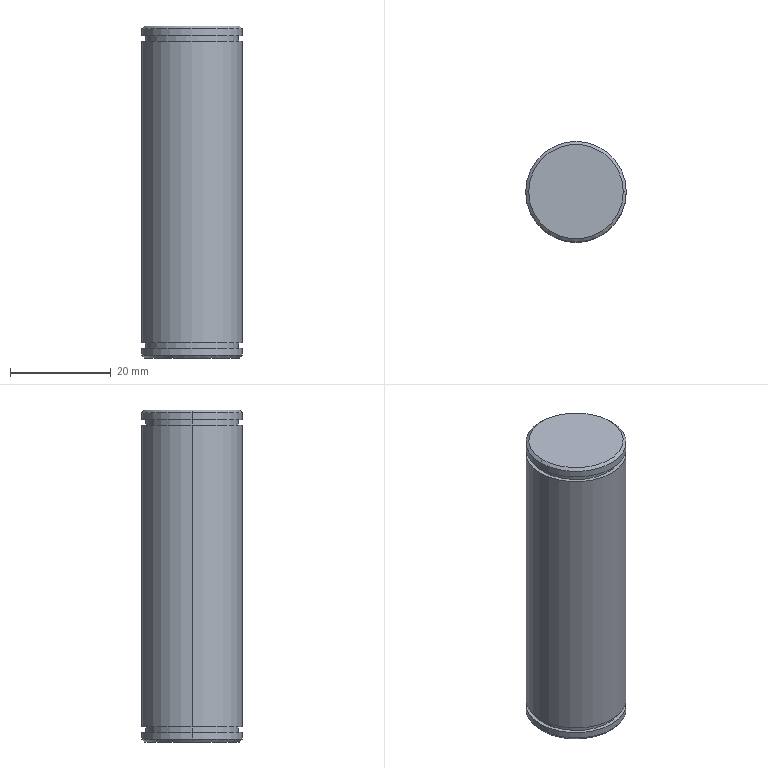Component | SolidWorks | ConnectingPin1-1 | 1 solid | 20 faces | box 20 x 20 x 66 mm | volume 20616 mm3 | cylinder 10 | plane 6 | cone 4 | commonest cylinder face diameters 20 x6 18.5 x4
build123d program:
from build123d import *
from OCP.BRepFilletAPI import BRepFilletAPI_MakeChamfer

# Parameters (mm, degrees)
SKETCH1_R           = 10
BOSS_EXTRUDE1_DEPTH = 33
CHAMFER1_SIZE       = 0.5
CHAMFER1_SIZE2      = 0.5959
SKETCH3_W           = 0.75
SKETCH3_H           = 1.1


with BuildPart() as part:
    # Sketch1 → Boss-Extrude1 (new, symmetric)
    with BuildSketch(Plane.XY):
        Circle(SKETCH1_R)
    extrude(amount=BOSS_EXTRUDE1_DEPTH, both=True)

    # Chamfer1: one chamfer whose edges measure the first distance from different faces: ONE call of the kernel's chamfer builder (chamfer() names one face for all edges)
    chamfer1_edges_1 = [part.edges().sort_by_distance(p)[0] for p in [
        (-10, 0, -33),
    ]]
    chamfer1_side_1 = [part.faces().sort_by_distance(p)[0] for p in [
        (0, 0, -33),
    ]]
    chamfer1_edges_2 = [part.edges().sort_by_distance(p)[0] for p in [
        (-10, 0, 33),
    ]]
    chamfer1_side_2 = [part.faces().sort_by_distance(p)[0] for p in [
        (-10, 0, 0),
    ]]
    chamfer1 = BRepFilletAPI_MakeChamfer(part.part.solid().wrapped)
    for e in chamfer1_edges_1:
        chamfer1.Add(CHAMFER1_SIZE, CHAMFER1_SIZE2, e.wrapped, chamfer1_side_1[0].wrapped)  # the first distance lies on this face
    for e in chamfer1_edges_2:
        chamfer1.Add(CHAMFER1_SIZE, CHAMFER1_SIZE2, e.wrapped, chamfer1_side_2[0].wrapped)  # the first distance lies on this face
    add(Compound.cast(chamfer1.Shape()), mode=Mode.REPLACE)

    # Sketch3 → Cut-Revolve1 (revolve, cut)
    with BuildSketch(Plane(origin=(0, 0, 0), x_dir=(1, 0, 0), z_dir=(0, 1, 0))):
        with Locations((9.625, -30.55)):
            Rectangle(SKETCH3_W, SKETCH3_H)
    cut_revolve1 = revolve(axis=Axis((0, 0, 33), (0, 0, -1)), mode=Mode.SUBTRACT)

    # Mirror2: Cut-Revolve1 across plane
    add(cut_revolve1.mirror(Plane.XY), mode=Mode.SUBTRACT)


solid = part.part

# Placed as in the assembly
solid = solid.moved(Location((-372.766, -43.543, 900), (0, 0, 0)))
STEP:
#1=COLOUR_RGB('',0.7922,0.8196,0.9333);
#2=FILL_AREA_STYLE_COLOUR('',#1);
#3=FILL_AREA_STYLE('',(#2));
#4=SURFACE_STYLE_FILL_AREA(#3);
#5=SURFACE_SIDE_STYLE('',(#4));
#6=SURFACE_STYLE_USAGE(.BOTH.,#5);
#7=PRESENTATION_STYLE_ASSIGNMENT((#6));
#8=CARTESIAN_POINT('',(-14.282,-1.714,34.209));
#9=VERTEX_POINT('',#8);
#10=CARTESIAN_POINT('',(-15.07,-1.714,34.209));
#11=VERTEX_POINT('',#10);
#12=CARTESIAN_POINT('',(-14.676,-1.714,34.209));
#13=DIRECTION('',(0.,-0.,1.));
#14=DIRECTION('',(1.,0.,0.));
#15=AXIS2_PLACEMENT_3D('',#12,#13,#14);
#16=CIRCLE('',#15,0.3937);
#17=EDGE_CURVE('',#9,#11,#16,.T.);
#18=ORIENTED_EDGE('',*,*,#17,.F.);
#19=CARTESIAN_POINT('',(-14.282,-1.714,34.157));
#20=VERTEX_POINT('',#19);
#21=CARTESIAN_POINT('',(-14.282,-1.714,36.732));
#22=DIRECTION('',(-0.,0.,-1.));
#23=VECTOR('',#22,39.37);
#24=LINE('',#21,#23);
#25=EDGE_CURVE('',#9,#20,#24,.T.);
#26=ORIENTED_EDGE('',*,*,#25,.T.);
#27=CARTESIAN_POINT('',(-15.07,-1.714,34.157));
#28=VERTEX_POINT('',#27);
#29=CARTESIAN_POINT('',(-14.676,-1.714,34.157));
#30=DIRECTION('',(0.,-0.,1.));
#31=DIRECTION('',(1.,0.,0.));
#32=AXIS2_PLACEMENT_3D('',#29,#30,#31);
#33=CIRCLE('',#32,0.3937);
#34=EDGE_CURVE('',#20,#28,#33,.T.);
#35=ORIENTED_EDGE('',*,*,#34,.T.);
#36=CARTESIAN_POINT('',(-15.07,-1.714,36.732));
#37=DIRECTION('',(-0.,0.,-1.));
#38=VECTOR('',#37,39.37);
#39=LINE('',#36,#38);
#40=EDGE_CURVE('',#11,#28,#39,.T.);
#41=ORIENTED_EDGE('',*,*,#40,.F.);
#42=EDGE_LOOP('',(#18,#26,#35,#41));
#43=FACE_OUTER_BOUND('',#42,.T.);
#44=CARTESIAN_POINT('',(-14.676,-1.714,36.732));
#45=DIRECTION('',(-0.,0.,-1.));
#46=DIRECTION('',(-1.,-0.,0.));
#47=AXIS2_PLACEMENT_3D('',#44,#45,#46);
#48=CYLINDRICAL_SURFACE('',#47,0.3937);
#49=ADVANCED_FACE('',(#43),#48,.T.);
#50=CARTESIAN_POINT('',(-15.05,-1.714,34.134));
#51=VERTEX_POINT('',#50);
#52=CARTESIAN_POINT('',(-14.302,-1.714,34.134));
#53=VERTEX_POINT('',#52);
#54=CARTESIAN_POINT('',(-14.676,-1.714,34.134));
#55=DIRECTION('',(-0.,0.,-1.));
#56=DIRECTION('',(1.,0.,0.));
#57=AXIS2_PLACEMENT_3D('',#54,#55,#56);
#58=CIRCLE('',#57,0.374);
#59=EDGE_CURVE('',#51,#53,#58,.T.);
#60=ORIENTED_EDGE('',*,*,#59,.F.);
#61=CARTESIAN_POINT('',(-15.07,-1.714,34.157));
#62=DIRECTION('',(-0.6428,-0.,0.766));
#63=VECTOR('',#62,39.37);
#64=LINE('',#61,#63);
#65=EDGE_CURVE('',#51,#28,#64,.T.);
#66=ORIENTED_EDGE('',*,*,#65,.T.);
#67=ORIENTED_EDGE('',*,*,#34,.F.);
#68=CARTESIAN_POINT('',(-14.282,-1.714,34.157));
#69=DIRECTION('',(0.6428,0.,0.766));
#70=VECTOR('',#69,39.37);
#71=LINE('',#68,#70);
#72=EDGE_CURVE('',#53,#20,#71,.T.);
#73=ORIENTED_EDGE('',*,*,#72,.F.);
#74=EDGE_LOOP('',(#60,#66,#67,#73));
#75=FACE_OUTER_BOUND('',#74,.T.);
#76=CARTESIAN_POINT('',(-14.676,-1.714,34.157));
#77=DIRECTION('',(0.,-0.,1.));
#78=DIRECTION('',(1.,0.,0.));
#79=AXIS2_PLACEMENT_3D('',#76,#77,#78);
#80=CONICAL_SURFACE('',#79,0.3937,0.6981);
#81=ADVANCED_FACE('',(#75),#80,.T.);
#82=CARTESIAN_POINT('',(-15.04,-1.714,34.252));
#83=VERTEX_POINT('',#82);
#84=CARTESIAN_POINT('',(-14.312,-1.714,34.252));
#85=VERTEX_POINT('',#84);
#86=CARTESIAN_POINT('',(-14.676,-1.714,34.252));
#87=DIRECTION('',(0.,-0.,1.));
#88=DIRECTION('',(1.,0.,0.));
#89=AXIS2_PLACEMENT_3D('',#86,#87,#88);
#90=CIRCLE('',#89,0.3642);
#91=EDGE_CURVE('',#83,#85,#90,.T.);
#92=ORIENTED_EDGE('',*,*,#91,.F.);
#93=CARTESIAN_POINT('',(-15.04,-1.714,34.209));
#94=VERTEX_POINT('',#93);
#95=CARTESIAN_POINT('',(-15.04,-1.714,34.252));
#96=DIRECTION('',(-0.,0.,-1.));
#97=VECTOR('',#96,39.37);
#98=LINE('',#95,#97);
#99=EDGE_CURVE('',#83,#94,#98,.T.);
#100=ORIENTED_EDGE('',*,*,#99,.T.);
#101=CARTESIAN_POINT('',(-14.312,-1.714,34.209));
#102=VERTEX_POINT('',#101);
#103=CARTESIAN_POINT('',(-14.676,-1.714,34.209));
#104=DIRECTION('',(0.,-0.,1.));
#105=DIRECTION('',(1.,0.,0.));
#106=AXIS2_PLACEMENT_3D('',#103,#104,#105);
#107=CIRCLE('',#106,0.3642);
#108=EDGE_CURVE('',#94,#102,#107,.T.);
#109=ORIENTED_EDGE('',*,*,#108,.T.);
#110=CARTESIAN_POINT('',(-14.312,-1.714,34.252));
#111=DIRECTION('',(-0.,0.,-1.));
#112=VECTOR('',#111,39.37);
#113=LINE('',#110,#112);
#114=EDGE_CURVE('',#85,#102,#113,.T.);
#115=ORIENTED_EDGE('',*,*,#114,.F.);
#116=EDGE_LOOP('',(#92,#100,#109,#115));
#117=FACE_OUTER_BOUND('',#116,.T.);
#118=CARTESIAN_POINT('',(-14.676,-1.714,34.252));
#119=DIRECTION('',(-0.,0.,-1.));
#120=DIRECTION('',(1.,0.,0.));
#121=AXIS2_PLACEMENT_3D('',#118,#119,#120);
#122=CYLINDRICAL_SURFACE('',#121,0.3642);
#123=ADVANCED_FACE('',(#117),#122,.T.);
#124=CARTESIAN_POINT('',(-15.07,-1.714,36.713));
#125=VERTEX_POINT('',#124);
#126=CARTESIAN_POINT('',(-14.282,-1.714,36.713));
#127=VERTEX_POINT('',#126);
#128=CARTESIAN_POINT('',(-14.676,-1.714,36.713));
#129=DIRECTION('',(-0.,0.,-1.));
#130=DIRECTION('',(1.,0.,0.));
#131=AXIS2_PLACEMENT_3D('',#128,#129,#130);
#132=CIRCLE('',#131,0.3937);
#133=EDGE_CURVE('',#125,#127,#132,.T.);
#134=ORIENTED_EDGE('',*,*,#133,.T.);
#135=CARTESIAN_POINT('',(-14.282,-1.714,36.657));
#136=VERTEX_POINT('',#135);
#137=CARTESIAN_POINT('',(-14.282,-1.714,36.732));
#138=DIRECTION('',(-0.,0.,-1.));
#139=VECTOR('',#138,39.37);
#140=LINE('',#137,#139);
#141=EDGE_CURVE('',#127,#136,#140,.T.);
#142=ORIENTED_EDGE('',*,*,#141,.T.);
#143=CARTESIAN_POINT('',(-15.07,-1.714,36.657));
#144=VERTEX_POINT('',#143);
#145=CARTESIAN_POINT('',(-14.676,-1.714,36.657));
#146=DIRECTION('',(0.,-0.,1.));
#147=DIRECTION('',(1.,0.,0.));
#148=AXIS2_PLACEMENT_3D('',#145,#146,#147);
#149=CIRCLE('',#148,0.3937);
#150=EDGE_CURVE('',#136,#144,#149,.T.);
#151=ORIENTED_EDGE('',*,*,#150,.T.);
#152=CARTESIAN_POINT('',(-15.07,-1.714,36.732));
#153=DIRECTION('',(-0.,0.,-1.));
#154=VECTOR('',#153,39.37);
#155=LINE('',#152,#154);
#156=EDGE_CURVE('',#125,#144,#155,.T.);
#157=ORIENTED_EDGE('',*,*,#156,.F.);
#158=EDGE_LOOP('',(#134,#142,#151,#157));
#159=FACE_OUTER_BOUND('',#158,.T.);
#160=CARTESIAN_POINT('',(-14.676,-1.714,36.732));
#161=DIRECTION('',(-0.,0.,-1.));
#162=DIRECTION('',(-1.,-0.,0.));
#163=AXIS2_PLACEMENT_3D('',#160,#161,#162);
#164=CYLINDRICAL_SURFACE('',#163,0.3937);
#165=ADVANCED_FACE('',(#159),#164,.T.);
#166=CARTESIAN_POINT('',(-14.306,-1.714,36.732));
#167=VERTEX_POINT('',#166);
#168=CARTESIAN_POINT('',(-15.046,-1.714,36.732));
#169=VERTEX_POINT('',#168);
#170=CARTESIAN_POINT('',(-14.676,-1.714,36.732));
#171=DIRECTION('',(0.,-0.,1.));
#172=DIRECTION('',(1.,0.,0.));
#173=AXIS2_PLACEMENT_3D('',#170,#171,#172);
#174=CIRCLE('',#173,0.3702);
#175=EDGE_CURVE('',#167,#169,#174,.T.);
#176=ORIENTED_EDGE('',*,*,#175,.F.);
#177=CARTESIAN_POINT('',(-14.306,-1.714,36.732));
#178=DIRECTION('',(0.766,0.,-0.6428));
#179=VECTOR('',#178,39.37);
#180=LINE('',#177,#179);
#181=EDGE_CURVE('',#167,#127,#180,.T.);
#182=ORIENTED_EDGE('',*,*,#181,.T.);
#183=ORIENTED_EDGE('',*,*,#133,.F.);
#184=CARTESIAN_POINT('',(-15.046,-1.714,36.732));
#185=DIRECTION('',(-0.766,-0.,-0.6428));
#186=VECTOR('',#185,39.37);
#187=LINE('',#184,#186);
#188=EDGE_CURVE('',#169,#125,#187,.T.);
#189=ORIENTED_EDGE('',*,*,#188,.F.);
#190=EDGE_LOOP('',(#176,#182,#183,#189));
#191=FACE_OUTER_BOUND('',#190,.T.);
#192=CARTESIAN_POINT('',(-14.676,-1.714,36.732));
#193=DIRECTION('',(-0.,0.,-1.));
#194=DIRECTION('',(-1.,-0.,0.));
#195=AXIS2_PLACEMENT_3D('',#192,#193,#194);
#196=CONICAL_SURFACE('',#195,0.3702,0.8727);
#197=ADVANCED_FACE('',(#191),#196,.T.);
#198=CARTESIAN_POINT('',(-14.312,-1.714,36.614));
#199=VERTEX_POINT('',#198);
#200=CARTESIAN_POINT('',(-15.04,-1.714,36.614));
#201=VERTEX_POINT('',#200);
#202=CARTESIAN_POINT('',(-14.676,-1.714,36.614));
#203=DIRECTION('',(0.,-0.,1.));
#204=DIRECTION('',(1.,0.,0.));
#205=AXIS2_PLACEMENT_3D('',#202,#203,#204);
#206=CIRCLE('',#205,0.3642);
#207=EDGE_CURVE('',#199,#201,#206,.T.);
#208=ORIENTED_EDGE('',*,*,#207,.T.);
#209=CARTESIAN_POINT('',(-15.04,-1.714,36.657));
#210=VERTEX_POINT('',#209);
#211=CARTESIAN_POINT('',(-15.04,-1.714,36.713));
#212=DIRECTION('',(0.,-0.,1.));
#213=VECTOR('',#212,39.37);
#214=LINE('',#211,#213);
#215=EDGE_CURVE('',#201,#210,#214,.T.);
#216=ORIENTED_EDGE('',*,*,#215,.T.);
#217=CARTESIAN_POINT('',(-14.312,-1.714,36.657));
#218=VERTEX_POINT('',#217);
#219=CARTESIAN_POINT('',(-14.676,-1.714,36.657));
#220=DIRECTION('',(0.,-0.,1.));
#221=DIRECTION('',(1.,0.,0.));
#222=AXIS2_PLACEMENT_3D('',#219,#220,#221);
#223=CIRCLE('',#222,0.3642);
#224=EDGE_CURVE('',#218,#210,#223,.T.);
#225=ORIENTED_EDGE('',*,*,#224,.F.);
#226=CARTESIAN_POINT('',(-14.312,-1.714,36.713));
#227=DIRECTION('',(0.,-0.,1.));
#228=VECTOR('',#227,39.37);
#229=LINE('',#226,#228);
#230=EDGE_CURVE('',#199,#218,#229,.T.);
#231=ORIENTED_EDGE('',*,*,#230,.F.);
#232=EDGE_LOOP('',(#208,#216,#225,#231));
#233=FACE_OUTER_BOUND('',#232,.T.);
#234=CARTESIAN_POINT('',(-14.676,-1.714,36.713));
#235=DIRECTION('',(0.,-0.,1.));
#236=DIRECTION('',(1.,0.,0.));
#237=AXIS2_PLACEMENT_3D('',#234,#235,#236);
#238=CYLINDRICAL_SURFACE('',#237,0.3642);
#239=ADVANCED_FACE('',(#233),#238,.T.);
#240=CARTESIAN_POINT('',(-14.282,-1.714,36.614));
#241=VERTEX_POINT('',#240);
#242=CARTESIAN_POINT('',(-15.07,-1.714,36.614));
#243=VERTEX_POINT('',#242);
#244=CARTESIAN_POINT('',(-14.676,-1.714,36.614));
#245=DIRECTION('',(0.,-0.,1.));
#246=DIRECTION('',(1.,0.,0.));
#247=AXIS2_PLACEMENT_3D('',#244,#245,#246);
#248=CIRCLE('',#247,0.3937);
#249=EDGE_CURVE('',#241,#243,#248,.T.);
#250=ORIENTED_EDGE('',*,*,#249,.F.);
#251=CARTESIAN_POINT('',(-14.282,-1.714,34.252));
#252=VERTEX_POINT('',#251);
#253=CARTESIAN_POINT('',(-14.282,-1.714,36.732));
#254=DIRECTION('',(-0.,0.,-1.));
#255=VECTOR('',#254,39.37);
#256=LINE('',#253,#255);
#257=EDGE_CURVE('',#241,#252,#256,.T.);
#258=ORIENTED_EDGE('',*,*,#257,.T.);
#259=CARTESIAN_POINT('',(-15.07,-1.714,34.252));
#260=VERTEX_POINT('',#259);
#261=CARTESIAN_POINT('',(-14.676,-1.714,34.252));
#262=DIRECTION('',(0.,-0.,1.));
#263=DIRECTION('',(1.,0.,0.));
#264=AXIS2_PLACEMENT_3D('',#261,#262,#263);
#265=CIRCLE('',#264,0.3937);
#266=EDGE_CURVE('',#252,#260,#265,.T.);
#267=ORIENTED_EDGE('',*,*,#266,.T.);
#268=CARTESIAN_POINT('',(-15.07,-1.714,36.732));
#269=DIRECTION('',(-0.,0.,-1.));
#270=VECTOR('',#269,39.37);
#271=LINE('',#268,#270);
#272=EDGE_CURVE('',#243,#260,#271,.T.);
#273=ORIENTED_EDGE('',*,*,#272,.F.);
#274=EDGE_LOOP('',(#250,#258,#267,#273));
#275=FACE_OUTER_BOUND('',#274,.T.);
#276=CARTESIAN_POINT('',(-14.676,-1.714,36.732));
#277=DIRECTION('',(-0.,0.,-1.));
#278=DIRECTION('',(-1.,-0.,0.));
#279=AXIS2_PLACEMENT_3D('',#276,#277,#278);
#280=CYLINDRICAL_SURFACE('',#279,0.3937);
#281=ADVANCED_FACE('',(#275),#280,.T.);
#282=ORIENTED_EDGE('',*,*,#257,.F.);
#283=CARTESIAN_POINT('',(-14.676,-1.714,36.614));
#284=DIRECTION('',(0.,-0.,1.));
#285=DIRECTION('',(1.,0.,0.));
#286=AXIS2_PLACEMENT_3D('',#283,#284,#285);
#287=CIRCLE('',#286,0.3937);
#288=EDGE_CURVE('',#243,#241,#287,.T.);
#289=ORIENTED_EDGE('',*,*,#288,.F.);
#290=ORIENTED_EDGE('',*,*,#272,.T.);
#291=CARTESIAN_POINT('',(-14.676,-1.714,34.252));
#292=DIRECTION('',(0.,-0.,1.));
#293=DIRECTION('',(1.,0.,0.));
#294=AXIS2_PLACEMENT_3D('',#291,#292,#293);
#295=CIRCLE('',#294,0.3937);
#296=EDGE_CURVE('',#260,#252,#295,.T.);
#297=ORIENTED_EDGE('',*,*,#296,.T.);
#298=EDGE_LOOP('',(#282,#289,#290,#297));
#299=FACE_OUTER_BOUND('',#298,.T.);
#300=CARTESIAN_POINT('',(-14.676,-1.714,36.732));
#301=DIRECTION('',(-0.,0.,-1.));
#302=DIRECTION('',(-1.,-0.,0.));
#303=AXIS2_PLACEMENT_3D('',#300,#301,#302);
#304=CYLINDRICAL_SURFACE('',#303,0.3937);
#305=ADVANCED_FACE('',(#299),#304,.T.);
#306=ORIENTED_EDGE('',*,*,#207,.F.);
#307=CARTESIAN_POINT('',(-14.676,-1.714,36.614));
#308=DIRECTION('',(0.,-0.,1.));
#309=DIRECTION('',(1.,0.,0.));
#310=AXIS2_PLACEMENT_3D('',#307,#308,#309);
#311=CIRCLE('',#310,0.3642);
#312=EDGE_CURVE('',#201,#199,#311,.T.);
#313=ORIENTED_EDGE('',*,*,#312,.F.);
#314=EDGE_LOOP('',(#306,#313));
#315=FACE_BOUND('',#314,.T.);
#316=ORIENTED_EDGE('',*,*,#288,.T.);
#317=ORIENTED_EDGE('',*,*,#249,.T.);
#318=EDGE_LOOP('',(#316,#317));
#319=FACE_OUTER_BOUND('',#318,.T.);
#320=CARTESIAN_POINT('',(-14.282,-1.714,36.614));
#321=DIRECTION('',(-0.,0.,-1.));
#322=DIRECTION('',(-1.,-0.,0.));
#323=AXIS2_PLACEMENT_3D('',#320,#321,#322);
#324=PLANE('',#323);
#325=ADVANCED_FACE('',(#315,#319),#324,.F.);
#326=ORIENTED_EDGE('',*,*,#215,.F.);
#327=ORIENTED_EDGE('',*,*,#312,.T.);
#328=ORIENTED_EDGE('',*,*,#230,.T.);
#329=CARTESIAN_POINT('',(-14.676,-1.714,36.657));
#330=DIRECTION('',(0.,-0.,1.));
#331=DIRECTION('',(1.,0.,0.));
#332=AXIS2_PLACEMENT_3D('',#329,#330,#331);
#333=CIRCLE('',#332,0.3642);
#334=EDGE_CURVE('',#210,#218,#333,.T.);
#335=ORIENTED_EDGE('',*,*,#334,.F.);
#336=EDGE_LOOP('',(#326,#327,#328,#335));
#337=FACE_OUTER_BOUND('',#336,.T.);
#338=CARTESIAN_POINT('',(-14.676,-1.714,36.713));
#339=DIRECTION('',(0.,-0.,1.));
#340=DIRECTION('',(1.,0.,0.));
#341=AXIS2_PLACEMENT_3D('',#338,#339,#340);
#342=CYLINDRICAL_SURFACE('',#341,0.3642);
#343=ADVANCED_FACE('',(#337),#342,.T.);
#344=CARTESIAN_POINT('',(-14.676,-1.714,36.657));
#345=DIRECTION('',(0.,-0.,1.));
#346=DIRECTION('',(1.,0.,0.));
#347=AXIS2_PLACEMENT_3D('',#344,#345,#346);
#348=CIRCLE('',#347,0.3937);
#349=EDGE_CURVE('',#144,#136,#348,.T.);
#350=ORIENTED_EDGE('',*,*,#349,.F.);
#351=ORIENTED_EDGE('',*,*,#150,.F.);
#352=EDGE_LOOP('',(#350,#351));
#353=FACE_OUTER_BOUND('',#352,.T.);
#354=ORIENTED_EDGE('',*,*,#224,.T.);
#355=ORIENTED_EDGE('',*,*,#334,.T.);
#356=EDGE_LOOP('',(#354,#355));
#357=FACE_BOUND('',#356,.T.);
#358=CARTESIAN_POINT('',(-14.282,-1.714,36.657));
#359=DIRECTION('',(0.,-0.,1.));
#360=DIRECTION('',(1.,0.,-0.));
#361=AXIS2_PLACEMENT_3D('',#358,#359,#360);
#362=PLANE('',#361);
#363=ADVANCED_FACE('',(#353,#357),#362,.F.);
#364=CARTESIAN_POINT('',(-14.676,-1.714,36.732));
#365=DIRECTION('',(0.,-0.,1.));
#366=DIRECTION('',(1.,0.,0.));
#367=AXIS2_PLACEMENT_3D('',#364,#365,#366);
#368=CIRCLE('',#367,0.3702);
#369=EDGE_CURVE('',#169,#167,#368,.T.);
#370=ORIENTED_EDGE('',*,*,#369,.T.);
#371=ORIENTED_EDGE('',*,*,#175,.T.);
#372=EDGE_LOOP('',(#370,#371));
#373=FACE_OUTER_BOUND('',#372,.T.);
#374=CARTESIAN_POINT('',(-14.676,-1.714,36.732));
#375=DIRECTION('',(0.,-0.,1.));
#376=DIRECTION('',(1.,0.,-0.));
#377=AXIS2_PLACEMENT_3D('',#374,#375,#376);
#378=PLANE('',#377);
#379=ADVANCED_FACE('',(#373),#378,.T.);
#380=ORIENTED_EDGE('',*,*,#181,.F.);
#381=ORIENTED_EDGE('',*,*,#369,.F.);
#382=ORIENTED_EDGE('',*,*,#188,.T.);
#383=CARTESIAN_POINT('',(-14.676,-1.714,36.713));
#384=DIRECTION('',(-0.,0.,-1.));
#385=DIRECTION('',(1.,0.,0.));
#386=AXIS2_PLACEMENT_3D('',#383,#384,#385);
#387=CIRCLE('',#386,0.3937);
#388=EDGE_CURVE('',#127,#125,#387,.T.);
#389=ORIENTED_EDGE('',*,*,#388,.F.);
#390=EDGE_LOOP('',(#380,#381,#382,#389));
#391=FACE_OUTER_BOUND('',#390,.T.);
#392=CARTESIAN_POINT('',(-14.676,-1.714,36.732));
#393=DIRECTION('',(-0.,0.,-1.));
#394=DIRECTION('',(-1.,-0.,0.));
#395=AXIS2_PLACEMENT_3D('',#392,#393,#394);
#396=CONICAL_SURFACE('',#395,0.3702,0.8727);
#397=ADVANCED_FACE('',(#391),#396,.T.);
#398=ORIENTED_EDGE('',*,*,#141,.F.);
#399=ORIENTED_EDGE('',*,*,#388,.T.);
#400=ORIENTED_EDGE('',*,*,#156,.T.);
#401=ORIENTED_EDGE('',*,*,#349,.T.);
#402=EDGE_LOOP('',(#398,#399,#400,#401));
#403=FACE_OUTER_BOUND('',#402,.T.);
#404=CARTESIAN_POINT('',(-14.676,-1.714,36.732));
#405=DIRECTION('',(-0.,0.,-1.));
#406=DIRECTION('',(-1.,-0.,0.));
#407=AXIS2_PLACEMENT_3D('',#404,#405,#406);
#408=CYLINDRICAL_SURFACE('',#407,0.3937);
#409=ADVANCED_FACE('',(#403),#408,.T.);
#410=CARTESIAN_POINT('',(-14.676,-1.714,34.252));
#411=DIRECTION('',(0.,-0.,1.));
#412=DIRECTION('',(1.,0.,0.));
#413=AXIS2_PLACEMENT_3D('',#410,#411,#412);
#414=CIRCLE('',#413,0.3642);
#415=EDGE_CURVE('',#85,#83,#414,.T.);
#416=ORIENTED_EDGE('',*,*,#415,.T.);
#417=ORIENTED_EDGE('',*,*,#91,.T.);
#418=EDGE_LOOP('',(#416,#417));
#419=FACE_BOUND('',#418,.T.);
#420=ORIENTED_EDGE('',*,*,#296,.F.);
#421=ORIENTED_EDGE('',*,*,#266,.F.);
#422=EDGE_LOOP('',(#420,#421));
#423=FACE_OUTER_BOUND('',#422,.T.);
#424=CARTESIAN_POINT('',(-14.282,-1.714,34.252));
#425=DIRECTION('',(0.,-0.,1.));
#426=DIRECTION('',(-1.,-0.,0.));
#427=AXIS2_PLACEMENT_3D('',#424,#425,#426);
#428=PLANE('',#427);
#429=ADVANCED_FACE('',(#419,#423),#428,.F.);
#430=ORIENTED_EDGE('',*,*,#99,.F.);
#431=ORIENTED_EDGE('',*,*,#415,.F.);
#432=ORIENTED_EDGE('',*,*,#114,.T.);
#433=CARTESIAN_POINT('',(-14.676,-1.714,34.209));
#434=DIRECTION('',(0.,-0.,1.));
#435=DIRECTION('',(1.,0.,0.));
#436=AXIS2_PLACEMENT_3D('',#433,#434,#435);
#437=CIRCLE('',#436,0.3642);
#438=EDGE_CURVE('',#102,#94,#437,.T.);
#439=ORIENTED_EDGE('',*,*,#438,.T.);
#440=EDGE_LOOP('',(#430,#431,#432,#439));
#441=FACE_OUTER_BOUND('',#440,.T.);
#442=CARTESIAN_POINT('',(-14.676,-1.714,34.252));
#443=DIRECTION('',(-0.,0.,-1.));
#444=DIRECTION('',(1.,0.,0.));
#445=AXIS2_PLACEMENT_3D('',#442,#443,#444);
#446=CYLINDRICAL_SURFACE('',#445,0.3642);
#447=ADVANCED_FACE('',(#441),#446,.T.);
#448=CARTESIAN_POINT('',(-14.676,-1.714,34.209));
#449=DIRECTION('',(0.,-0.,1.));
#450=DIRECTION('',(1.,0.,0.));
#451=AXIS2_PLACEMENT_3D('',#448,#449,#450);
#452=CIRCLE('',#451,0.3937);
#453=EDGE_CURVE('',#11,#9,#452,.T.);
#454=ORIENTED_EDGE('',*,*,#453,.T.);
#455=ORIENTED_EDGE('',*,*,#17,.T.);
#456=EDGE_LOOP('',(#454,#455));
#457=FACE_OUTER_BOUND('',#456,.T.);
#458=ORIENTED_EDGE('',*,*,#438,.F.);
#459=ORIENTED_EDGE('',*,*,#108,.F.);
#460=EDGE_LOOP('',(#458,#459));
#461=FACE_BOUND('',#460,.T.);
#462=CARTESIAN_POINT('',(-14.282,-1.714,34.209));
#463=DIRECTION('',(-0.,0.,-1.));
#464=DIRECTION('',(1.,0.,-0.));
#465=AXIS2_PLACEMENT_3D('',#462,#463,#464);
#466=PLANE('',#465);
#467=ADVANCED_FACE('',(#457,#461),#466,.F.);
#468=CARTESIAN_POINT('',(-14.676,-1.714,34.134));
#469=DIRECTION('',(-0.,0.,-1.));
#470=DIRECTION('',(1.,0.,0.));
#471=AXIS2_PLACEMENT_3D('',#468,#469,#470);
#472=CIRCLE('',#471,0.374);
#473=EDGE_CURVE('',#53,#51,#472,.T.);
#474=ORIENTED_EDGE('',*,*,#473,.T.);
#475=ORIENTED_EDGE('',*,*,#59,.T.);
#476=EDGE_LOOP('',(#474,#475));
#477=FACE_OUTER_BOUND('',#476,.T.);
#478=CARTESIAN_POINT('',(-14.676,-1.714,34.134));
#479=DIRECTION('',(0.,-0.,1.));
#480=DIRECTION('',(1.,0.,-0.));
#481=AXIS2_PLACEMENT_3D('',#478,#479,#480);
#482=PLANE('',#481);
#483=ADVANCED_FACE('',(#477),#482,.F.);
#484=ORIENTED_EDGE('',*,*,#65,.F.);
#485=ORIENTED_EDGE('',*,*,#473,.F.);
#486=ORIENTED_EDGE('',*,*,#72,.T.);
#487=CARTESIAN_POINT('',(-14.676,-1.714,34.157));
#488=DIRECTION('',(0.,-0.,1.));
#489=DIRECTION('',(1.,0.,0.));
#490=AXIS2_PLACEMENT_3D('',#487,#488,#489);
#491=CIRCLE('',#490,0.3937);
#492=EDGE_CURVE('',#28,#20,#491,.T.);
#493=ORIENTED_EDGE('',*,*,#492,.F.);
#494=EDGE_LOOP('',(#484,#485,#486,#493));
#495=FACE_OUTER_BOUND('',#494,.T.);
#496=CARTESIAN_POINT('',(-14.676,-1.714,34.157));
#497=DIRECTION('',(0.,-0.,1.));
#498=DIRECTION('',(1.,0.,0.));
#499=AXIS2_PLACEMENT_3D('',#496,#497,#498);
#500=CONICAL_SURFACE('',#499,0.3937,0.6981);
#501=ADVANCED_FACE('',(#495),#500,.T.);
#502=ORIENTED_EDGE('',*,*,#25,.F.);
#503=ORIENTED_EDGE('',*,*,#453,.F.);
#504=ORIENTED_EDGE('',*,*,#40,.T.);
#505=ORIENTED_EDGE('',*,*,#492,.T.);
#506=EDGE_LOOP('',(#502,#503,#504,#505));
#507=FACE_OUTER_BOUND('',#506,.T.);
#508=CARTESIAN_POINT('',(-14.676,-1.714,36.732));
#509=DIRECTION('',(-0.,0.,-1.));
#510=DIRECTION('',(-1.,-0.,0.));
#511=AXIS2_PLACEMENT_3D('',#508,#509,#510);
#512=CYLINDRICAL_SURFACE('',#511,0.3937);
#513=ADVANCED_FACE('',(#507),#512,.T.);
#514=CLOSED_SHELL('',(#49,#81,#123,#165,#197,#239,#281,#305,#325,#343,#363,#379,#397,#409,#429,#447,#467,#483,#501,#513));
#515=MANIFOLD_SOLID_BREP('',#514);
#516=STYLED_ITEM('',(#7),#515);
#517=PRESENTATION_LAYER_ASSIGNMENT('','',(#516));
#518=(LENGTH_UNIT()NAMED_UNIT(*)SI_UNIT($,.METRE.));
#519=LENGTH_MEASURE_WITH_UNIT(LENGTH_MEASURE(0.0254),#518);
#520=DIMENSIONAL_EXPONENTS(1.,0.,0.,0.,0.,0.,0.);
#521=(CONVERSION_BASED_UNIT('',#519)LENGTH_UNIT()NAMED_UNIT(#520));
#522=UNCERTAINTY_MEASURE_WITH_UNIT(LENGTH_MEASURE(0.00001),#521,'','');
#523=(NAMED_UNIT(*)PLANE_ANGLE_UNIT()SI_UNIT($,.RADIAN.));
#524=(NAMED_UNIT(*)SI_UNIT($,.STERADIAN.)SOLID_ANGLE_UNIT());
#525=(GEOMETRIC_REPRESENTATION_CONTEXT(3)GLOBAL_UNCERTAINTY_ASSIGNED_CONTEXT((#522))GLOBAL_UNIT_ASSIGNED_CONTEXT((#521,#523,#524))REPRESENTATION_CONTEXT('',''));
#526=MECHANICAL_DESIGN_GEOMETRIC_PRESENTATION_REPRESENTATION('',(#516),#525);
#527=CARTESIAN_POINT('',(0.,0.,0.));
#528=DIRECTION('',(0.,0.,1.));
#529=DIRECTION('',(1.,0.,0.));
#530=AXIS2_PLACEMENT_3D('',#527,#528,#529);
#531=(LENGTH_UNIT()NAMED_UNIT(*)SI_UNIT($,.METRE.));
#532=LENGTH_MEASURE_WITH_UNIT(LENGTH_MEASURE(0.0254),#531);
#533=DIMENSIONAL_EXPONENTS(1.,0.,0.,0.,0.,0.,0.);
#534=(CONVERSION_BASED_UNIT('',#532)LENGTH_UNIT()NAMED_UNIT(#533));
#535=UNCERTAINTY_MEASURE_WITH_UNIT(LENGTH_MEASURE(0.00001),#534,'','');
#536=(NAMED_UNIT(*)PLANE_ANGLE_UNIT()SI_UNIT($,.RADIAN.));
#537=(NAMED_UNIT(*)SI_UNIT($,.STERADIAN.)SOLID_ANGLE_UNIT());
#538=(GEOMETRIC_REPRESENTATION_CONTEXT(3)GLOBAL_UNCERTAINTY_ASSIGNED_CONTEXT((#535))GLOBAL_UNIT_ASSIGNED_CONTEXT((#534,#536,#537))REPRESENTATION_CONTEXT('',''));
#539=ADVANCED_BREP_SHAPE_REPRESENTATION('',(#515,#530),#538);